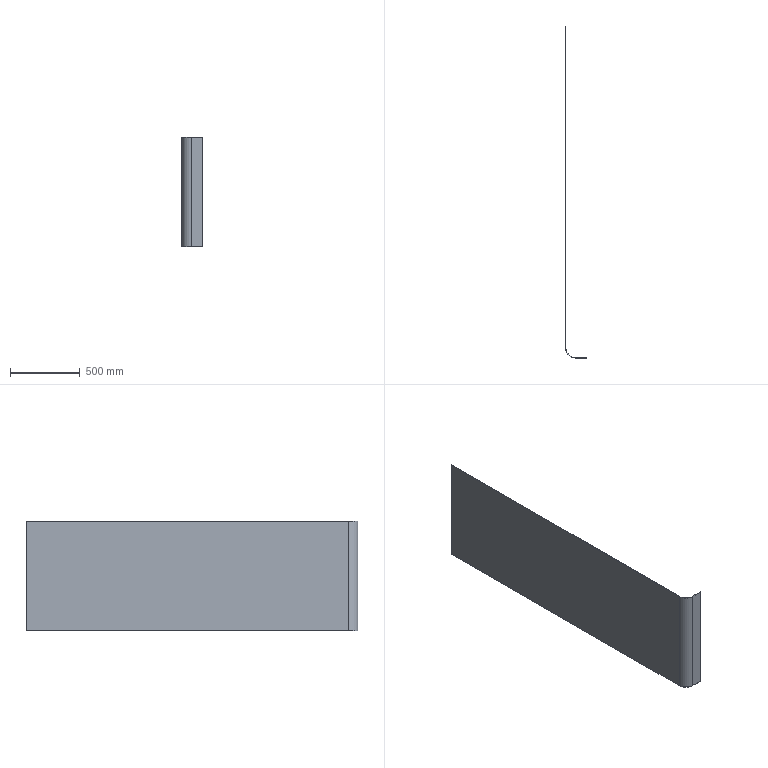Component | SolidWorks | D-SideAluminumHousingAssembly-1_D-SideAluminumCasing-1 | 1 solid | 14 faces | box 149.5 x 2375.5 x 782 mm | volume 5848142 mm3 | plane 12 | cylinder 2 | commonest cylinder face diameters 139 x1 133 x1
STEP:
#1=COLOUR_RGB('',0.7922,0.8196,0.9333);
#2=FILL_AREA_STYLE_COLOUR('',#1);
#3=FILL_AREA_STYLE('',(#2));
#4=SURFACE_STYLE_FILL_AREA(#3);
#5=SURFACE_SIDE_STYLE('',(#4));
#6=SURFACE_STYLE_USAGE(.BOTH.,#5);
#7=PRESENTATION_STYLE_ASSIGNMENT((#6));
#8=CARTESIAN_POINT('',(-39.862,-0.,67.815));
#9=VERTEX_POINT('',#8);
#10=CARTESIAN_POINT('',(-39.98,-0.,67.815));
#11=VERTEX_POINT('',#10);
#12=CARTESIAN_POINT('',(-39.98,-0.,67.815));
#13=DIRECTION('',(-1.,-0.,-0.));
#14=VECTOR('',#13,39.37);
#15=LINE('',#12,#14);
#16=EDGE_CURVE('',#9,#11,#15,.T.);
#17=ORIENTED_EDGE('',*,*,#16,.F.);
#18=CARTESIAN_POINT('',(-39.862,90.787,67.815));
#19=VERTEX_POINT('',#18);
#20=CARTESIAN_POINT('',(-39.862,-0.,67.815));
#21=DIRECTION('',(-0.,1.,0.));
#22=VECTOR('',#21,39.37);
#23=LINE('',#20,#22);
#24=EDGE_CURVE('',#9,#19,#23,.T.);
#25=ORIENTED_EDGE('',*,*,#24,.T.);
#26=CARTESIAN_POINT('',(-39.98,90.787,67.815));
#27=VERTEX_POINT('',#26);
#28=CARTESIAN_POINT('',(-39.98,90.787,67.815));
#29=DIRECTION('',(-1.,-0.,-0.));
#30=VECTOR('',#29,39.37);
#31=LINE('',#28,#30);
#32=EDGE_CURVE('',#19,#27,#31,.T.);
#33=ORIENTED_EDGE('',*,*,#32,.T.);
#34=CARTESIAN_POINT('',(-39.98,-0.,67.815));
#35=DIRECTION('',(-0.,1.,0.));
#36=VECTOR('',#35,39.37);
#37=LINE('',#34,#36);
#38=EDGE_CURVE('',#11,#27,#37,.T.);
#39=ORIENTED_EDGE('',*,*,#38,.F.);
#40=EDGE_LOOP('',(#17,#25,#33,#39));
#41=FACE_OUTER_BOUND('',#40,.T.);
#42=CARTESIAN_POINT('',(-39.98,-0.,67.815));
#43=DIRECTION('',(0.,0.,-1.));
#44=DIRECTION('',(-0.,1.,0.));
#45=AXIS2_PLACEMENT_3D('',#42,#43,#44);
#46=PLANE('',#45);
#47=ADVANCED_FACE('',(#41),#46,.F.);
#48=ORIENTED_EDGE('',*,*,#32,.F.);
#49=CARTESIAN_POINT('',(-39.862,90.787,37.028));
#50=VERTEX_POINT('',#49);
#51=CARTESIAN_POINT('',(-39.862,90.787,37.028));
#52=DIRECTION('',(0.,0.,-1.));
#53=VECTOR('',#52,39.37);
#54=LINE('',#51,#53);
#55=EDGE_CURVE('',#19,#50,#54,.T.);
#56=ORIENTED_EDGE('',*,*,#55,.T.);
#57=CARTESIAN_POINT('',(-39.98,90.787,37.028));
#58=VERTEX_POINT('',#57);
#59=CARTESIAN_POINT('',(-39.98,90.787,37.028));
#60=DIRECTION('',(-1.,-0.,-0.));
#61=VECTOR('',#60,39.37);
#62=LINE('',#59,#61);
#63=EDGE_CURVE('',#50,#58,#62,.T.);
#64=ORIENTED_EDGE('',*,*,#63,.T.);
#65=CARTESIAN_POINT('',(-39.98,90.787,37.028));
#66=DIRECTION('',(0.,0.,-1.));
#67=VECTOR('',#66,39.37);
#68=LINE('',#65,#67);
#69=EDGE_CURVE('',#27,#58,#68,.T.);
#70=ORIENTED_EDGE('',*,*,#69,.F.);
#71=EDGE_LOOP('',(#48,#56,#64,#70));
#72=FACE_OUTER_BOUND('',#71,.T.);
#73=CARTESIAN_POINT('',(-39.98,90.787,37.028));
#74=DIRECTION('',(0.,-1.,-0.));
#75=DIRECTION('',(0.,0.,-1.));
#76=AXIS2_PLACEMENT_3D('',#73,#74,#75);
#77=PLANE('',#76);
#78=ADVANCED_FACE('',(#72),#77,.F.);
#79=ORIENTED_EDGE('',*,*,#63,.F.);
#80=CARTESIAN_POINT('',(-39.862,-0.,37.028));
#81=VERTEX_POINT('',#80);
#82=CARTESIAN_POINT('',(-39.862,-0.,37.028));
#83=DIRECTION('',(0.,-1.,-0.));
#84=VECTOR('',#83,39.37);
#85=LINE('',#82,#84);
#86=EDGE_CURVE('',#50,#81,#85,.T.);
#87=ORIENTED_EDGE('',*,*,#86,.T.);
#88=CARTESIAN_POINT('',(-39.98,-0.,37.028));
#89=VERTEX_POINT('',#88);
#90=CARTESIAN_POINT('',(-39.98,-0.,37.028));
#91=DIRECTION('',(-1.,-0.,-0.));
#92=VECTOR('',#91,39.37);
#93=LINE('',#90,#92);
#94=EDGE_CURVE('',#81,#89,#93,.T.);
#95=ORIENTED_EDGE('',*,*,#94,.T.);
#96=CARTESIAN_POINT('',(-39.98,-0.,37.028));
#97=DIRECTION('',(0.,-1.,-0.));
#98=VECTOR('',#97,39.37);
#99=LINE('',#96,#98);
#100=EDGE_CURVE('',#58,#89,#99,.T.);
#101=ORIENTED_EDGE('',*,*,#100,.F.);
#102=EDGE_LOOP('',(#79,#87,#95,#101));
#103=FACE_OUTER_BOUND('',#102,.T.);
#104=CARTESIAN_POINT('',(-39.98,-0.,37.028));
#105=DIRECTION('',(-0.,-0.,1.));
#106=DIRECTION('',(0.,-1.,-0.));
#107=AXIS2_PLACEMENT_3D('',#104,#105,#106);
#108=PLANE('',#107);
#109=ADVANCED_FACE('',(#103),#108,.F.);
#110=ORIENTED_EDGE('',*,*,#100,.T.);
#111=CARTESIAN_POINT('',(-39.98,-0.,37.028));
#112=DIRECTION('',(-0.,-0.,1.));
#113=VECTOR('',#112,39.37);
#114=LINE('',#111,#113);
#115=EDGE_CURVE('',#89,#11,#114,.T.);
#116=ORIENTED_EDGE('',*,*,#115,.T.);
#117=ORIENTED_EDGE('',*,*,#38,.T.);
#118=ORIENTED_EDGE('',*,*,#69,.T.);
#119=EDGE_LOOP('',(#110,#116,#117,#118));
#120=FACE_OUTER_BOUND('',#119,.T.);
#121=CARTESIAN_POINT('',(-39.98,-0.,37.028));
#122=DIRECTION('',(1.,0.,0.));
#123=DIRECTION('',(0.,0.,-1.));
#124=AXIS2_PLACEMENT_3D('',#121,#122,#123);
#125=PLANE('',#124);
#126=ADVANCED_FACE('',(#120),#125,.F.);
#127=ORIENTED_EDGE('',*,*,#86,.F.);
#128=ORIENTED_EDGE('',*,*,#55,.F.);
#129=ORIENTED_EDGE('',*,*,#24,.F.);
#130=CARTESIAN_POINT('',(-39.862,-0.,37.028));
#131=DIRECTION('',(-0.,-0.,1.));
#132=VECTOR('',#131,39.37);
#133=LINE('',#130,#132);
#134=EDGE_CURVE('',#81,#9,#133,.T.);
#135=ORIENTED_EDGE('',*,*,#134,.F.);
#136=EDGE_LOOP('',(#127,#128,#129,#135));
#137=FACE_OUTER_BOUND('',#136,.T.);
#138=CARTESIAN_POINT('',(-39.862,-0.,37.028));
#139=DIRECTION('',(1.,0.,0.));
#140=DIRECTION('',(0.,0.,-1.));
#141=AXIS2_PLACEMENT_3D('',#138,#139,#140);
#142=PLANE('',#141);
#143=ADVANCED_FACE('',(#137),#142,.T.);
#144=CARTESIAN_POINT('',(-37.244,-2.618,67.815));
#145=VERTEX_POINT('',#144);
#146=CARTESIAN_POINT('',(-37.244,-2.736,67.815));
#147=VERTEX_POINT('',#146);
#148=CARTESIAN_POINT('',(-37.244,-2.736,67.815));
#149=DIRECTION('',(0.,-1.,-0.));
#150=VECTOR('',#149,39.37);
#151=LINE('',#148,#150);
#152=EDGE_CURVE('',#145,#147,#151,.T.);
#153=ORIENTED_EDGE('',*,*,#152,.F.);
#154=CARTESIAN_POINT('',(-37.244,-0.,67.815));
#155=DIRECTION('',(-0.,-0.,1.));
#156=DIRECTION('',(-1.,-0.,-0.));
#157=AXIS2_PLACEMENT_3D('',#154,#155,#156);
#158=CIRCLE('',#157,2.618);
#159=EDGE_CURVE('',#9,#145,#158,.T.);
#160=ORIENTED_EDGE('',*,*,#159,.F.);
#161=ORIENTED_EDGE('',*,*,#16,.T.);
#162=CARTESIAN_POINT('',(-37.244,-0.,67.815));
#163=DIRECTION('',(-0.,-0.,1.));
#164=DIRECTION('',(-1.,-0.,-0.));
#165=AXIS2_PLACEMENT_3D('',#162,#163,#164);
#166=CIRCLE('',#165,2.736);
#167=EDGE_CURVE('',#11,#147,#166,.T.);
#168=ORIENTED_EDGE('',*,*,#167,.T.);
#169=EDGE_LOOP('',(#153,#160,#161,#168));
#170=FACE_OUTER_BOUND('',#169,.T.);
#171=CARTESIAN_POINT('',(-37.244,-0.,67.815));
#172=DIRECTION('',(-0.,-0.,1.));
#173=DIRECTION('',(1.,0.,0.));
#174=AXIS2_PLACEMENT_3D('',#171,#172,#173);
#175=PLANE('',#174);
#176=ADVANCED_FACE('',(#170),#175,.T.);
#177=CARTESIAN_POINT('',(-37.244,-2.618,37.028));
#178=VERTEX_POINT('',#177);
#179=CARTESIAN_POINT('',(-37.244,-0.,37.028));
#180=DIRECTION('',(0.,0.,-1.));
#181=DIRECTION('',(-1.,-0.,-0.));
#182=AXIS2_PLACEMENT_3D('',#179,#180,#181);
#183=CIRCLE('',#182,2.618);
#184=EDGE_CURVE('',#178,#81,#183,.T.);
#185=ORIENTED_EDGE('',*,*,#184,.F.);
#186=CARTESIAN_POINT('',(-37.244,-2.736,37.028));
#187=VERTEX_POINT('',#186);
#188=CARTESIAN_POINT('',(-37.244,-2.618,37.028));
#189=DIRECTION('',(0.,-1.,-0.));
#190=VECTOR('',#189,39.37);
#191=LINE('',#188,#190);
#192=EDGE_CURVE('',#178,#187,#191,.T.);
#193=ORIENTED_EDGE('',*,*,#192,.T.);
#194=CARTESIAN_POINT('',(-37.244,-0.,37.028));
#195=DIRECTION('',(0.,0.,-1.));
#196=DIRECTION('',(-1.,-0.,-0.));
#197=AXIS2_PLACEMENT_3D('',#194,#195,#196);
#198=CIRCLE('',#197,2.736);
#199=EDGE_CURVE('',#187,#89,#198,.T.);
#200=ORIENTED_EDGE('',*,*,#199,.T.);
#201=ORIENTED_EDGE('',*,*,#94,.F.);
#202=EDGE_LOOP('',(#185,#193,#200,#201));
#203=FACE_OUTER_BOUND('',#202,.T.);
#204=CARTESIAN_POINT('',(-37.244,-0.,37.028));
#205=DIRECTION('',(-0.,-0.,1.));
#206=DIRECTION('',(1.,0.,0.));
#207=AXIS2_PLACEMENT_3D('',#204,#205,#206);
#208=PLANE('',#207);
#209=ADVANCED_FACE('',(#203),#208,.F.);
#210=ORIENTED_EDGE('',*,*,#115,.F.);
#211=ORIENTED_EDGE('',*,*,#199,.F.);
#212=CARTESIAN_POINT('',(-37.244,-2.736,67.815));
#213=DIRECTION('',(-0.,-0.,1.));
#214=VECTOR('',#213,39.37);
#215=LINE('',#212,#214);
#216=EDGE_CURVE('',#187,#147,#215,.T.);
#217=ORIENTED_EDGE('',*,*,#216,.T.);
#218=ORIENTED_EDGE('',*,*,#167,.F.);
#219=EDGE_LOOP('',(#210,#211,#217,#218));
#220=FACE_OUTER_BOUND('',#219,.T.);
#221=CARTESIAN_POINT('',(-37.244,-0.,37.028));
#222=DIRECTION('',(0.,0.,-1.));
#223=DIRECTION('',(0.,-1.,-0.));
#224=AXIS2_PLACEMENT_3D('',#221,#222,#223);
#225=CYLINDRICAL_SURFACE('',#224,2.736);
#226=ADVANCED_FACE('',(#220),#225,.T.);
#227=ORIENTED_EDGE('',*,*,#134,.T.);
#228=ORIENTED_EDGE('',*,*,#159,.T.);
#229=CARTESIAN_POINT('',(-37.244,-2.618,67.815));
#230=DIRECTION('',(0.,0.,-1.));
#231=VECTOR('',#230,39.37);
#232=LINE('',#229,#231);
#233=EDGE_CURVE('',#145,#178,#232,.T.);
#234=ORIENTED_EDGE('',*,*,#233,.T.);
#235=ORIENTED_EDGE('',*,*,#184,.T.);
#236=EDGE_LOOP('',(#227,#228,#234,#235));
#237=FACE_OUTER_BOUND('',#236,.T.);
#238=CARTESIAN_POINT('',(-37.244,-0.,37.028));
#239=DIRECTION('',(0.,0.,-1.));
#240=DIRECTION('',(0.,-1.,-0.));
#241=AXIS2_PLACEMENT_3D('',#238,#239,#240);
#242=CYLINDRICAL_SURFACE('',#241,2.618);
#243=ADVANCED_FACE('',(#237),#242,.F.);
#244=ORIENTED_EDGE('',*,*,#192,.F.);
#245=CARTESIAN_POINT('',(-34.094,-2.618,37.028));
#246=VERTEX_POINT('',#245);
#247=CARTESIAN_POINT('',(-34.094,-2.618,37.028));
#248=DIRECTION('',(1.,0.,0.));
#249=VECTOR('',#248,39.37);
#250=LINE('',#247,#249);
#251=EDGE_CURVE('',#178,#246,#250,.T.);
#252=ORIENTED_EDGE('',*,*,#251,.T.);
#253=CARTESIAN_POINT('',(-34.094,-2.736,37.028));
#254=VERTEX_POINT('',#253);
#255=CARTESIAN_POINT('',(-34.094,-2.736,37.028));
#256=DIRECTION('',(-0.,1.,0.));
#257=VECTOR('',#256,39.37);
#258=LINE('',#255,#257);
#259=EDGE_CURVE('',#254,#246,#258,.T.);
#260=ORIENTED_EDGE('',*,*,#259,.F.);
#261=CARTESIAN_POINT('',(-39.862,-2.736,37.028));
#262=DIRECTION('',(1.,0.,0.));
#263=VECTOR('',#262,39.37);
#264=LINE('',#261,#263);
#265=EDGE_CURVE('',#187,#254,#264,.T.);
#266=ORIENTED_EDGE('',*,*,#265,.F.);
#267=EDGE_LOOP('',(#244,#252,#260,#266));
#268=FACE_OUTER_BOUND('',#267,.T.);
#269=CARTESIAN_POINT('',(-34.094,-2.736,37.028));
#270=DIRECTION('',(-0.,-0.,1.));
#271=DIRECTION('',(1.,0.,0.));
#272=AXIS2_PLACEMENT_3D('',#269,#270,#271);
#273=PLANE('',#272);
#274=ADVANCED_FACE('',(#268),#273,.F.);
#275=ORIENTED_EDGE('',*,*,#152,.T.);
#276=CARTESIAN_POINT('',(-34.094,-2.736,67.815));
#277=VERTEX_POINT('',#276);
#278=CARTESIAN_POINT('',(-39.862,-2.736,67.815));
#279=DIRECTION('',(-1.,-0.,-0.));
#280=VECTOR('',#279,39.37);
#281=LINE('',#278,#280);
#282=EDGE_CURVE('',#277,#147,#281,.T.);
#283=ORIENTED_EDGE('',*,*,#282,.F.);
#284=CARTESIAN_POINT('',(-34.094,-2.618,67.815));
#285=VERTEX_POINT('',#284);
#286=CARTESIAN_POINT('',(-34.094,-2.736,67.815));
#287=DIRECTION('',(-0.,1.,0.));
#288=VECTOR('',#287,39.37);
#289=LINE('',#286,#288);
#290=EDGE_CURVE('',#277,#285,#289,.T.);
#291=ORIENTED_EDGE('',*,*,#290,.T.);
#292=CARTESIAN_POINT('',(-39.862,-2.618,67.815));
#293=DIRECTION('',(-1.,-0.,-0.));
#294=VECTOR('',#293,39.37);
#295=LINE('',#292,#294);
#296=EDGE_CURVE('',#285,#145,#295,.T.);
#297=ORIENTED_EDGE('',*,*,#296,.T.);
#298=EDGE_LOOP('',(#275,#283,#291,#297));
#299=FACE_OUTER_BOUND('',#298,.T.);
#300=CARTESIAN_POINT('',(-39.862,-2.736,67.815));
#301=DIRECTION('',(0.,0.,-1.));
#302=DIRECTION('',(-1.,-0.,-0.));
#303=AXIS2_PLACEMENT_3D('',#300,#301,#302);
#304=PLANE('',#303);
#305=ADVANCED_FACE('',(#299),#304,.F.);
#306=ORIENTED_EDGE('',*,*,#216,.F.);
#307=ORIENTED_EDGE('',*,*,#265,.T.);
#308=CARTESIAN_POINT('',(-34.094,-2.736,37.028));
#309=DIRECTION('',(-0.,-0.,1.));
#310=VECTOR('',#309,39.37);
#311=LINE('',#308,#310);
#312=EDGE_CURVE('',#254,#277,#311,.T.);
#313=ORIENTED_EDGE('',*,*,#312,.T.);
#314=ORIENTED_EDGE('',*,*,#282,.T.);
#315=EDGE_LOOP('',(#306,#307,#313,#314));
#316=FACE_OUTER_BOUND('',#315,.T.);
#317=CARTESIAN_POINT('',(-39.862,-2.736,37.028));
#318=DIRECTION('',(-0.,1.,0.));
#319=DIRECTION('',(-1.,-0.,-0.));
#320=AXIS2_PLACEMENT_3D('',#317,#318,#319);
#321=PLANE('',#320);
#322=ADVANCED_FACE('',(#316),#321,.F.);
#323=ORIENTED_EDGE('',*,*,#251,.F.);
#324=ORIENTED_EDGE('',*,*,#233,.F.);
#325=ORIENTED_EDGE('',*,*,#296,.F.);
#326=CARTESIAN_POINT('',(-34.094,-2.618,67.815));
#327=DIRECTION('',(-0.,-0.,1.));
#328=VECTOR('',#327,39.37);
#329=LINE('',#326,#328);
#330=EDGE_CURVE('',#246,#285,#329,.T.);
#331=ORIENTED_EDGE('',*,*,#330,.F.);
#332=EDGE_LOOP('',(#323,#324,#325,#331));
#333=FACE_OUTER_BOUND('',#332,.T.);
#334=CARTESIAN_POINT('',(-39.862,-2.618,37.028));
#335=DIRECTION('',(-0.,1.,0.));
#336=DIRECTION('',(-1.,-0.,-0.));
#337=AXIS2_PLACEMENT_3D('',#334,#335,#336);
#338=PLANE('',#337);
#339=ADVANCED_FACE('',(#333),#338,.T.);
#340=ORIENTED_EDGE('',*,*,#330,.T.);
#341=ORIENTED_EDGE('',*,*,#290,.F.);
#342=ORIENTED_EDGE('',*,*,#312,.F.);
#343=ORIENTED_EDGE('',*,*,#259,.T.);
#344=EDGE_LOOP('',(#340,#341,#342,#343));
#345=FACE_OUTER_BOUND('',#344,.T.);
#346=CARTESIAN_POINT('',(-34.094,-2.736,67.815));
#347=DIRECTION('',(-1.,0.,-0.));
#348=DIRECTION('',(0.,-1.,-0.));
#349=AXIS2_PLACEMENT_3D('',#346,#347,#348);
#350=PLANE('',#349);
#351=ADVANCED_FACE('',(#345),#350,.F.);
#352=CLOSED_SHELL('',(#47,#78,#109,#126,#143,#176,#209,#226,#243,#274,#305,#322,#339,#351));
#353=MANIFOLD_SOLID_BREP('',#352);
#354=STYLED_ITEM('',(#7),#353);
#355=PRESENTATION_LAYER_ASSIGNMENT('','',(#354));
#356=(LENGTH_UNIT()NAMED_UNIT(*)SI_UNIT($,.METRE.));
#357=LENGTH_MEASURE_WITH_UNIT(LENGTH_MEASURE(0.0254),#356);
#358=DIMENSIONAL_EXPONENTS(1.,0.,0.,0.,0.,0.,0.);
#359=(CONVERSION_BASED_UNIT('',#357)LENGTH_UNIT()NAMED_UNIT(#358));
#360=UNCERTAINTY_MEASURE_WITH_UNIT(LENGTH_MEASURE(0.00001),#359,'','');
#361=(NAMED_UNIT(*)PLANE_ANGLE_UNIT()SI_UNIT($,.RADIAN.));
#362=(NAMED_UNIT(*)SI_UNIT($,.STERADIAN.)SOLID_ANGLE_UNIT());
#363=(GEOMETRIC_REPRESENTATION_CONTEXT(3)GLOBAL_UNCERTAINTY_ASSIGNED_CONTEXT((#360))GLOBAL_UNIT_ASSIGNED_CONTEXT((#359,#361,#362))REPRESENTATION_CONTEXT('',''));
#364=MECHANICAL_DESIGN_GEOMETRIC_PRESENTATION_REPRESENTATION('',(#354),#363);
#365=CARTESIAN_POINT('',(0.,0.,0.));
#366=DIRECTION('',(0.,0.,1.));
#367=DIRECTION('',(1.,0.,0.));
#368=AXIS2_PLACEMENT_3D('',#365,#366,#367);
#369=(LENGTH_UNIT()NAMED_UNIT(*)SI_UNIT($,.METRE.));
#370=LENGTH_MEASURE_WITH_UNIT(LENGTH_MEASURE(0.0254),#369);
#371=DIMENSIONAL_EXPONENTS(1.,0.,0.,0.,0.,0.,0.);
#372=(CONVERSION_BASED_UNIT('',#370)LENGTH_UNIT()NAMED_UNIT(#371));
#373=UNCERTAINTY_MEASURE_WITH_UNIT(LENGTH_MEASURE(0.00001),#372,'','');
#374=(NAMED_UNIT(*)PLANE_ANGLE_UNIT()SI_UNIT($,.RADIAN.));
#375=(NAMED_UNIT(*)SI_UNIT($,.STERADIAN.)SOLID_ANGLE_UNIT());
#376=(GEOMETRIC_REPRESENTATION_CONTEXT(3)GLOBAL_UNCERTAINTY_ASSIGNED_CONTEXT((#373))GLOBAL_UNIT_ASSIGNED_CONTEXT((#372,#374,#375))REPRESENTATION_CONTEXT('',''));
#377=ADVANCED_BREP_SHAPE_REPRESENTATION('',(#353,#368),#376);